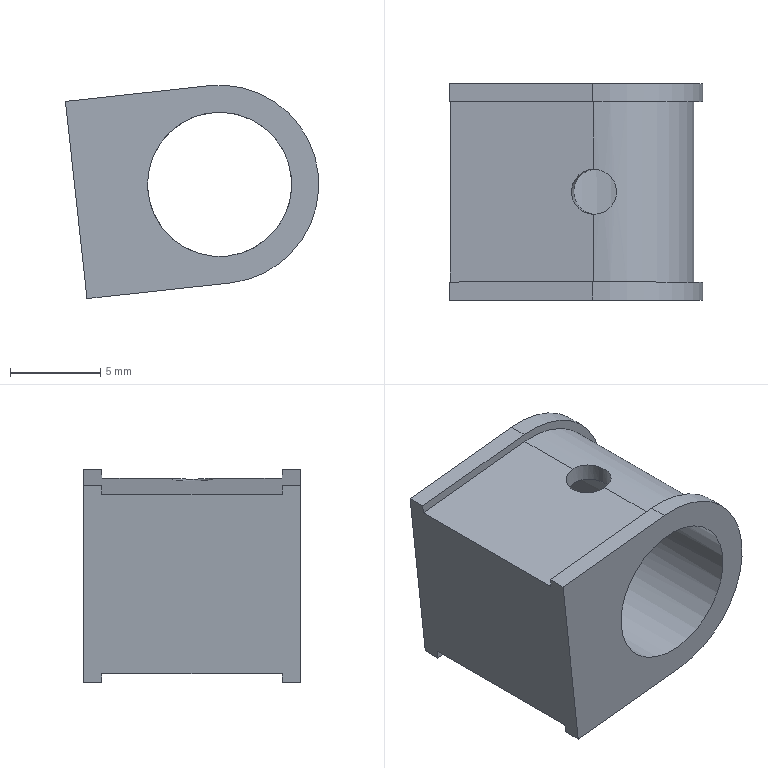Component | NX | LINK_3_LARGE_BLOCK | 1 solid | 16 faces | volume 855 mm3 | plane 11 | cylinder 5 | commonest cylinder face diameters 11 x2 10 x1 8 x1 2.5 x1